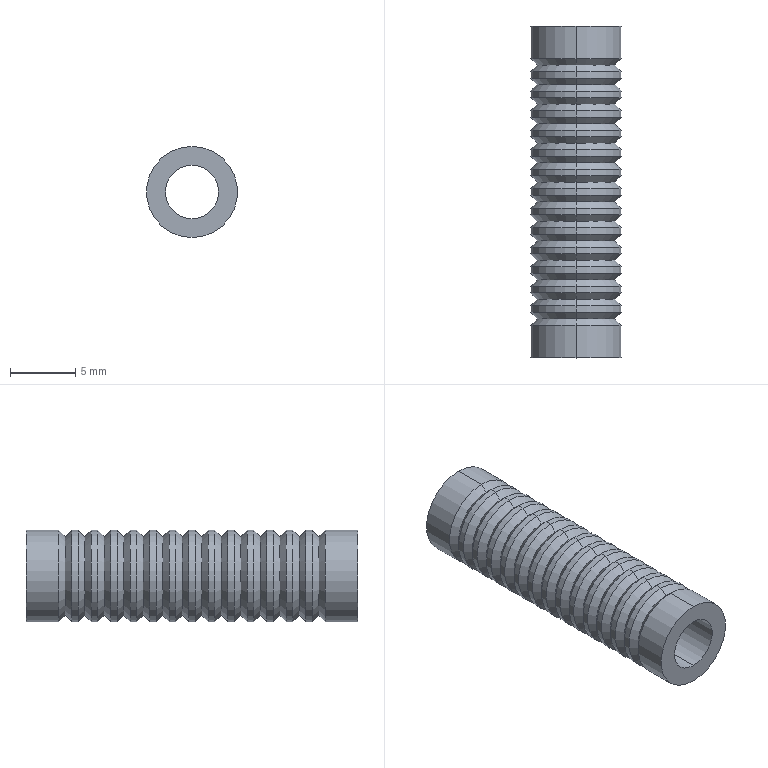Component | SolidWorks | 30604270309Roller-1 | 1 solid | 90 faces | box 7 x 25.5 x 7 mm | volume 571 mm3 | cone 56 | cylinder 32 | plane 2 | commonest cylinder face diameters 7 x30 4.1 x2 | material Teflon
build123d program:
from build123d import *

# Parameters (mm, degrees)
SKETCH1_R       = 3.5
SKETCH1_R_2     = 2.05
EXTRUDE1_DEPTH  = 12.75
LPATTERN1_COUNT = 14
LPATTERN1_PITCH = 1.5


with BuildPart() as part:
    # Sketch1 → Extrude1 (new, symmetric)
    with BuildSketch(Plane(origin=(0, 0, 0), x_dir=(0, 0, -1), z_dir=(1, 0, 0))):
        Circle(SKETCH1_R)
        Circle(SKETCH1_R_2, mode=Mode.SUBTRACT)
    extrude(amount=EXTRUDE1_DEPTH, both=True)

    # Sketch8 → Cut-Revolve6 (revolve, cut)
    with BuildSketch(Plane(origin=(0, 0, 0), x_dir=(1, 0, 0), z_dir=(0, 1, 0)), mode=Mode.PRIVATE) as cut_revolve6_sk:
        Polygon((9.25, 3.5), (9.75, 3), (10.25, 3.5), align=None)
    cut_revolve6 = revolve(cut_revolve6_sk.sketch.rotate(Axis((0, 0, 0), (1, 0, 0)), 180), axis=Axis((0, 0, 0), (1, 0, 0)), mode=Mode.SUBTRACT)

    # LPattern1: Cut-Revolve6 ×14
    with Locations(*[(-i * LPATTERN1_PITCH, 0, 0) for i in range(1, LPATTERN1_COUNT)]):
        add(cut_revolve6, mode=Mode.SUBTRACT)


solid = part.part

# Placed as in the assembly
solid = solid.moved(Location((210.87, 43.668, 34.729), (0, 0, 90)))